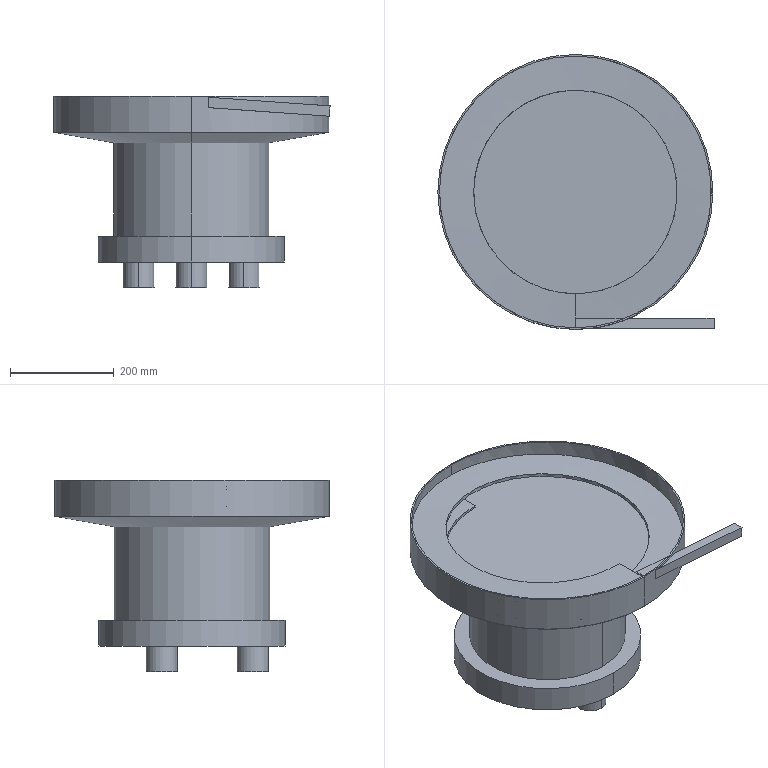Component | SolidWorks | PlasticVibratoryFeederCSFA2082-1 | 1 solid | 42 faces | volume 23006208 mm3 | plane 20 | cylinder 17 | spline 3 | cone 2 | commonest cylinder face diameters 60 x6 524 x5 300 x2 360 x2 530 x2